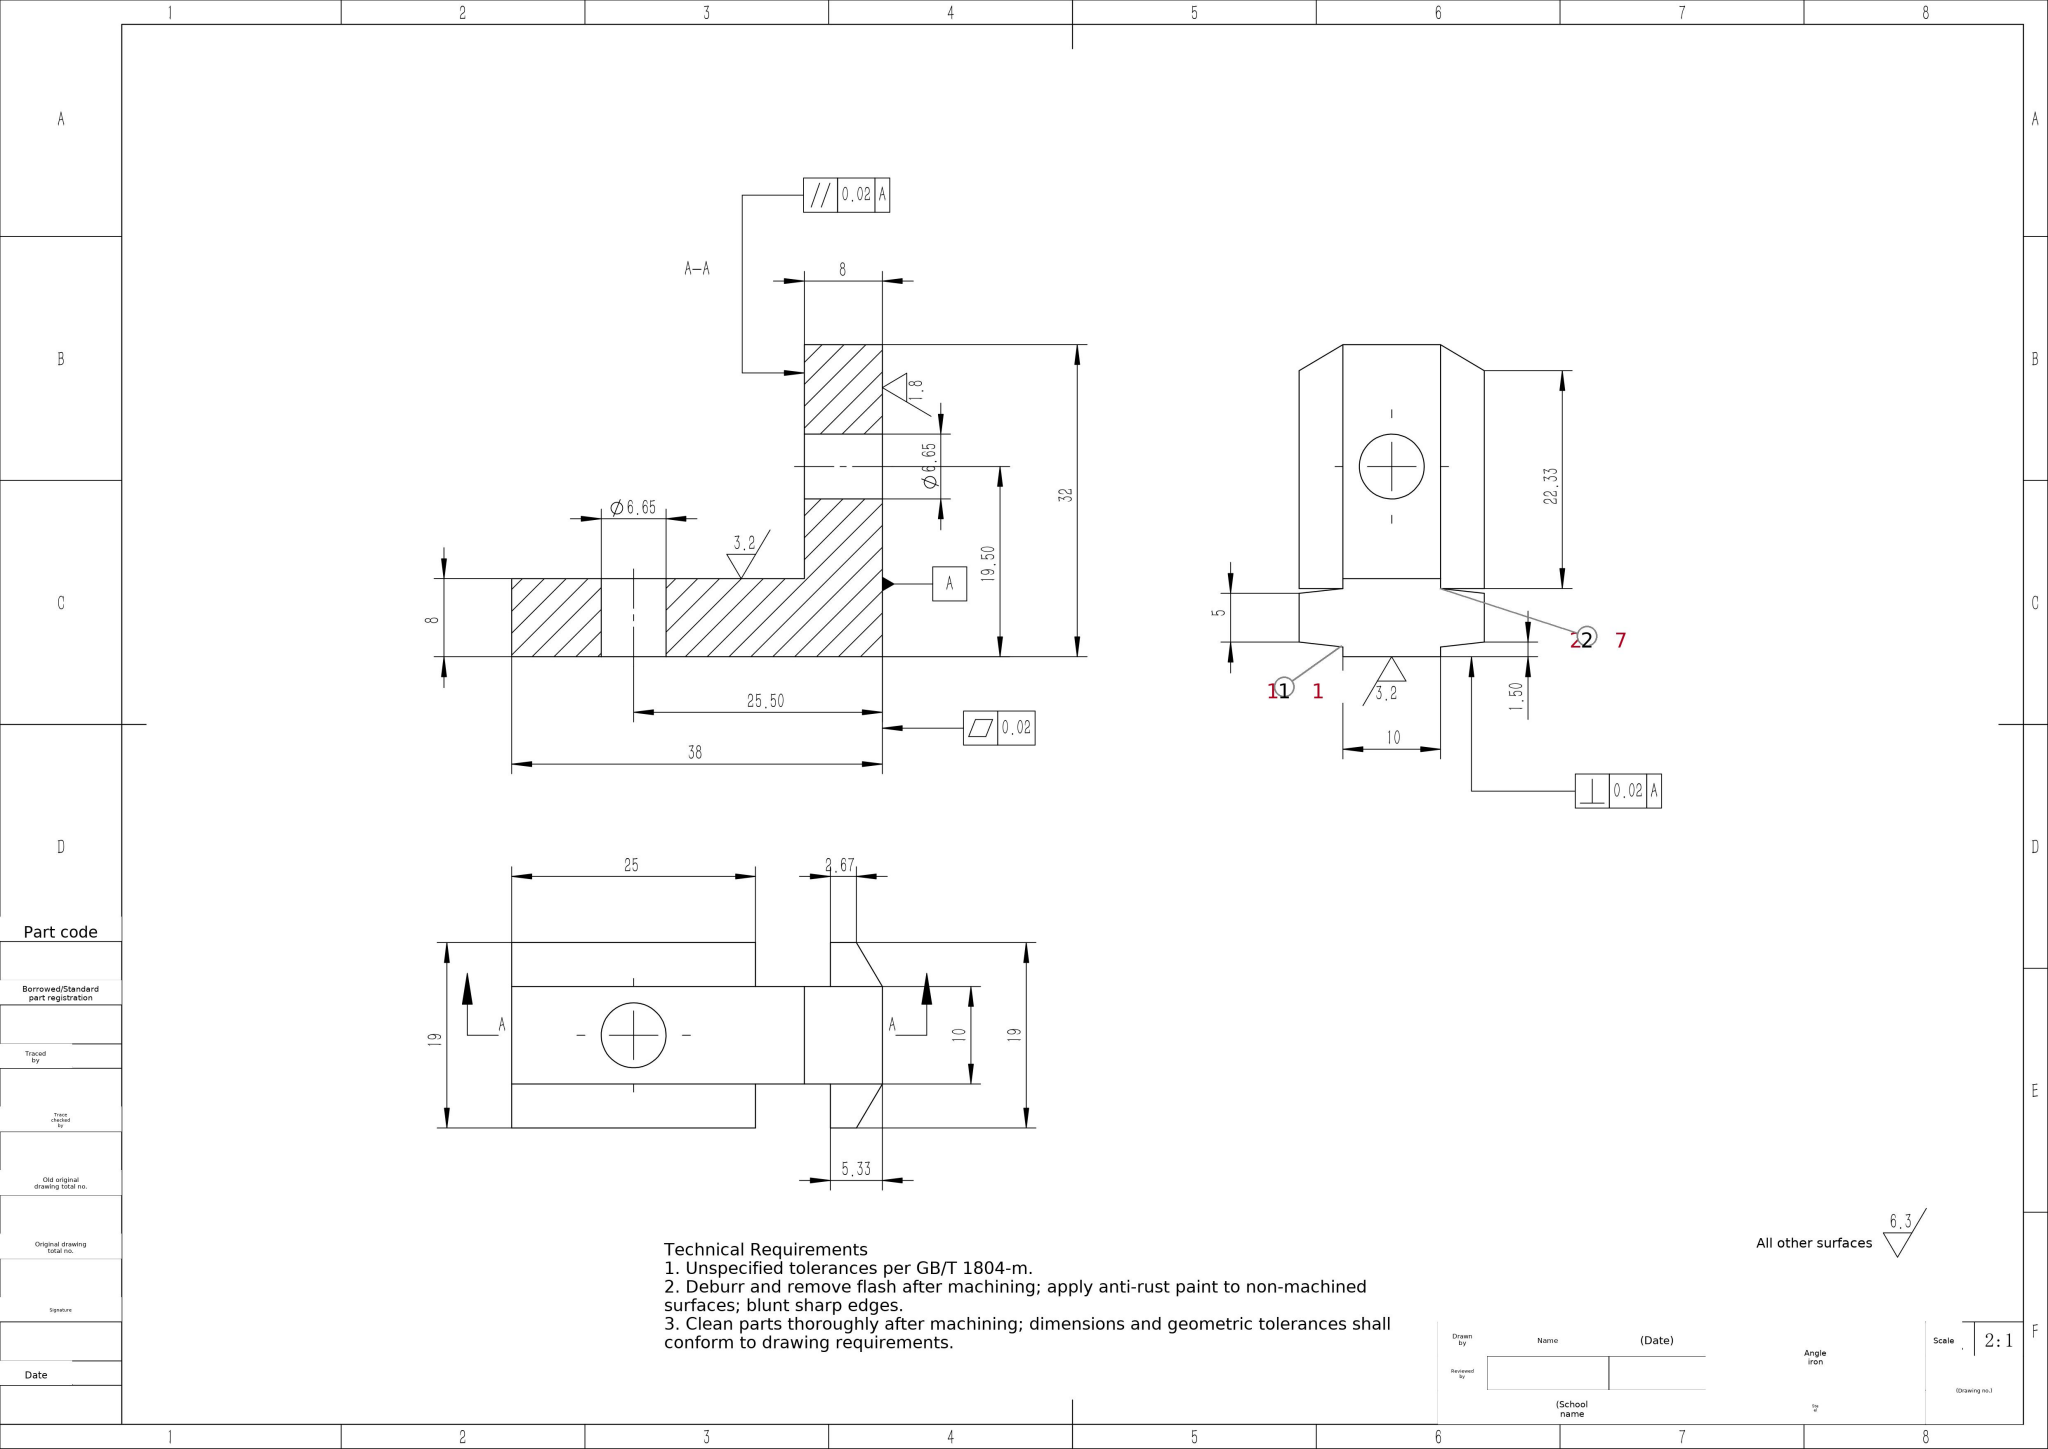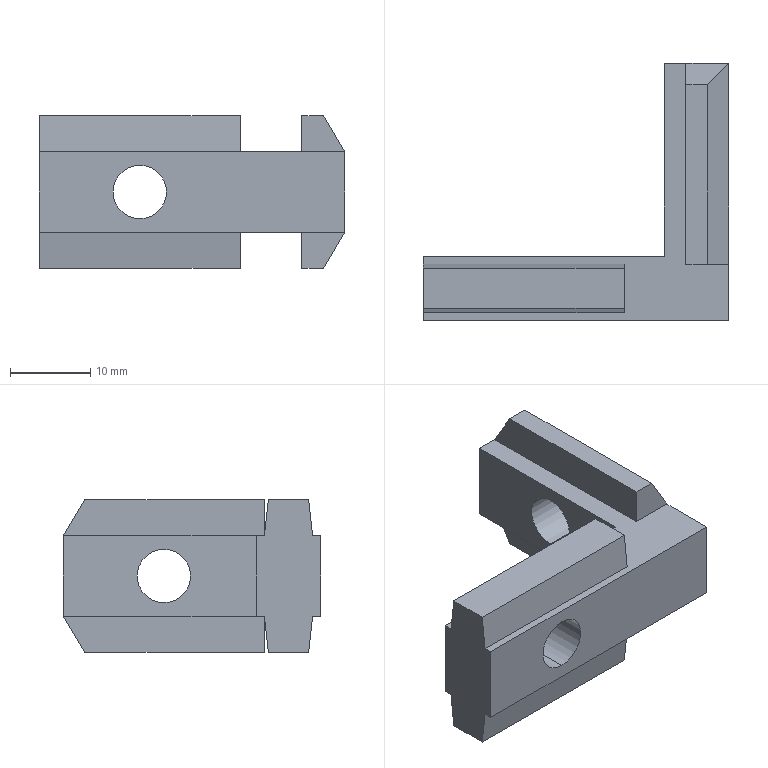Part | SolidWorks | mm | 1 solid | 30 faces | box 38 x 32 x 19 mm | volume 6500 mm3 | plane 26 | cylinder 4 | commonest cylinder face diameters 6.647 x4
STEP:
#1=CARTESIAN_POINT('',(0.,19.5,-3.324));
#2=VERTEX_POINT('',#1);
#3=CARTESIAN_POINT('',(0.,19.5,3.323));
#4=VERTEX_POINT('',#3);
#5=CARTESIAN_POINT('',(0.,19.5,-0.));
#6=DIRECTION('',(-1.,0.,0.));
#7=DIRECTION('',(0.,0.,1.));
#8=AXIS2_PLACEMENT_3D('',#5,#6,#7);
#9=CIRCLE('',#8,3.323);
#10=EDGE_CURVE('',#2,#4,#9,.T.);
#11=ORIENTED_EDGE('',*,*,#10,.F.);
#12=CARTESIAN_POINT('',(-8.,19.5,-3.323));
#13=VERTEX_POINT('',#12);
#14=CARTESIAN_POINT('',(-8.,19.5,-3.323));
#15=DIRECTION('',(-1.,0.,0.));
#16=VECTOR('',#15,1000.);
#17=LINE('',#14,#16);
#18=EDGE_CURVE('',#2,#13,#17,.T.);
#19=ORIENTED_EDGE('',*,*,#18,.T.);
#20=CARTESIAN_POINT('',(-8.,19.5,3.323));
#21=VERTEX_POINT('',#20);
#22=CARTESIAN_POINT('',(-8.,19.5,0.));
#23=DIRECTION('',(-1.,0.,0.));
#24=DIRECTION('',(0.,0.,1.));
#25=AXIS2_PLACEMENT_3D('',#22,#23,#24);
#26=CIRCLE('',#25,3.323);
#27=EDGE_CURVE('',#13,#21,#26,.T.);
#28=ORIENTED_EDGE('',*,*,#27,.T.);
#29=CARTESIAN_POINT('',(-8.,19.5,3.323));
#30=DIRECTION('',(-1.,0.,0.));
#31=VECTOR('',#30,1000.);
#32=LINE('',#29,#31);
#33=EDGE_CURVE('',#4,#21,#32,.T.);
#34=ORIENTED_EDGE('',*,*,#33,.F.);
#35=EDGE_LOOP('',(#11,#19,#28,#34));
#36=FACE_OUTER_BOUND('',#35,.T.);
#37=CARTESIAN_POINT('',(-8.,19.5,0.));
#38=DIRECTION('',(-1.,0.,0.));
#39=DIRECTION('',(0.,0.,1.));
#40=AXIS2_PLACEMENT_3D('',#37,#38,#39);
#41=CYLINDRICAL_SURFACE('',#40,3.323);
#42=ADVANCED_FACE('',(#36),#41,.F.);
#43=CARTESIAN_POINT('',(-25.5,8.,3.323));
#44=VERTEX_POINT('',#43);
#45=CARTESIAN_POINT('',(-25.5,8.,-3.323));
#46=VERTEX_POINT('',#45);
#47=CARTESIAN_POINT('',(-25.5,8.,0.));
#48=DIRECTION('',(-0.,-1.,-0.));
#49=DIRECTION('',(0.,0.,-1.));
#50=AXIS2_PLACEMENT_3D('',#47,#48,#49);
#51=CIRCLE('',#50,3.323);
#52=EDGE_CURVE('',#44,#46,#51,.T.);
#53=ORIENTED_EDGE('',*,*,#52,.F.);
#54=CARTESIAN_POINT('',(-25.5,-0.,3.323));
#55=VERTEX_POINT('',#54);
#56=CARTESIAN_POINT('',(-25.5,0.,3.323));
#57=DIRECTION('',(0.,-1.,0.));
#58=VECTOR('',#57,1000.);
#59=LINE('',#56,#58);
#60=EDGE_CURVE('',#44,#55,#59,.T.);
#61=ORIENTED_EDGE('',*,*,#60,.T.);
#62=CARTESIAN_POINT('',(-25.5,-0.,-3.323));
#63=VERTEX_POINT('',#62);
#64=CARTESIAN_POINT('',(-25.5,-0.,0.));
#65=DIRECTION('',(0.,-1.,0.));
#66=DIRECTION('',(0.,0.,-1.));
#67=AXIS2_PLACEMENT_3D('',#64,#65,#66);
#68=CIRCLE('',#67,3.323);
#69=EDGE_CURVE('',#55,#63,#68,.T.);
#70=ORIENTED_EDGE('',*,*,#69,.T.);
#71=CARTESIAN_POINT('',(-25.5,0.,-3.323));
#72=DIRECTION('',(0.,-1.,0.));
#73=VECTOR('',#72,1000.);
#74=LINE('',#71,#73);
#75=EDGE_CURVE('',#46,#63,#74,.T.);
#76=ORIENTED_EDGE('',*,*,#75,.F.);
#77=EDGE_LOOP('',(#53,#61,#70,#76));
#78=FACE_OUTER_BOUND('',#77,.T.);
#79=CARTESIAN_POINT('',(-25.5,0.,0.));
#80=DIRECTION('',(0.,-1.,0.));
#81=DIRECTION('',(0.,0.,-1.));
#82=AXIS2_PLACEMENT_3D('',#79,#80,#81);
#83=CYLINDRICAL_SURFACE('',#82,3.323);
#84=ADVANCED_FACE('',(#78),#83,.F.);
#85=CARTESIAN_POINT('',(0.,7.,-5.));
#86=VERTEX_POINT('',#85);
#87=CARTESIAN_POINT('',(-5.333,7.,-5.));
#88=VERTEX_POINT('',#87);
#89=CARTESIAN_POINT('',(-5.333,7.,-5.));
#90=DIRECTION('',(-1.,0.,0.));
#91=VECTOR('',#90,1000.);
#92=LINE('',#89,#91);
#93=EDGE_CURVE('',#86,#88,#92,.T.);
#94=ORIENTED_EDGE('',*,*,#93,.F.);
#95=CARTESIAN_POINT('',(0.,0.,-5.));
#96=VERTEX_POINT('',#95);
#97=CARTESIAN_POINT('',(0.,32.,-5.));
#98=DIRECTION('',(0.,-1.,-0.));
#99=VECTOR('',#98,1000.);
#100=LINE('',#97,#99);
#101=EDGE_CURVE('',#86,#96,#100,.T.);
#102=ORIENTED_EDGE('',*,*,#101,.T.);
#103=CARTESIAN_POINT('',(-38.,0.,-5.));
#104=VERTEX_POINT('',#103);
#105=CARTESIAN_POINT('',(0.,0.,-5.));
#106=DIRECTION('',(1.,0.,0.));
#107=VECTOR('',#106,1000.);
#108=LINE('',#105,#107);
#109=EDGE_CURVE('',#104,#96,#108,.T.);
#110=ORIENTED_EDGE('',*,*,#109,.F.);
#111=CARTESIAN_POINT('',(-38.,1.,-5.));
#112=VERTEX_POINT('',#111);
#113=CARTESIAN_POINT('',(-38.,0.,-5.));
#114=DIRECTION('',(0.,1.,0.));
#115=VECTOR('',#114,1000.);
#116=LINE('',#113,#115);
#117=EDGE_CURVE('',#104,#112,#116,.T.);
#118=ORIENTED_EDGE('',*,*,#117,.T.);
#119=CARTESIAN_POINT('',(-13.,1.,-5.));
#120=VERTEX_POINT('',#119);
#121=CARTESIAN_POINT('',(-38.,1.,-5.));
#122=DIRECTION('',(1.,0.,0.));
#123=VECTOR('',#122,1000.);
#124=LINE('',#121,#123);
#125=EDGE_CURVE('',#112,#120,#124,.T.);
#126=ORIENTED_EDGE('',*,*,#125,.T.);
#127=CARTESIAN_POINT('',(-13.,7.,-5.));
#128=VERTEX_POINT('',#127);
#129=CARTESIAN_POINT('',(-13.,7.,-5.));
#130=DIRECTION('',(0.,-1.,0.));
#131=VECTOR('',#130,1000.);
#132=LINE('',#129,#131);
#133=EDGE_CURVE('',#128,#120,#132,.T.);
#134=ORIENTED_EDGE('',*,*,#133,.F.);
#135=CARTESIAN_POINT('',(-38.,7.,-5.));
#136=VERTEX_POINT('',#135);
#137=CARTESIAN_POINT('',(-38.,7.,-5.));
#138=DIRECTION('',(1.,0.,0.));
#139=VECTOR('',#138,1000.);
#140=LINE('',#137,#139);
#141=EDGE_CURVE('',#136,#128,#140,.T.);
#142=ORIENTED_EDGE('',*,*,#141,.F.);
#143=CARTESIAN_POINT('',(-38.,8.,-5.));
#144=VERTEX_POINT('',#143);
#145=CARTESIAN_POINT('',(-38.,32.,-5.));
#146=DIRECTION('',(0.,-1.,-0.));
#147=VECTOR('',#146,1000.);
#148=LINE('',#145,#147);
#149=EDGE_CURVE('',#144,#136,#148,.T.);
#150=ORIENTED_EDGE('',*,*,#149,.F.);
#151=CARTESIAN_POINT('',(-8.,8.,-5.));
#152=VERTEX_POINT('',#151);
#153=CARTESIAN_POINT('',(-8.,8.,-5.));
#154=DIRECTION('',(-1.,0.,0.));
#155=VECTOR('',#154,1000.);
#156=LINE('',#153,#155);
#157=EDGE_CURVE('',#152,#144,#156,.T.);
#158=ORIENTED_EDGE('',*,*,#157,.F.);
#159=CARTESIAN_POINT('',(-8.,32.,-5.));
#160=VERTEX_POINT('',#159);
#161=CARTESIAN_POINT('',(-8.,32.,-5.));
#162=DIRECTION('',(0.,-1.,-0.));
#163=VECTOR('',#162,1000.);
#164=LINE('',#161,#163);
#165=EDGE_CURVE('',#160,#152,#164,.T.);
#166=ORIENTED_EDGE('',*,*,#165,.F.);
#167=CARTESIAN_POINT('',(-5.333,32.,-5.));
#168=VERTEX_POINT('',#167);
#169=CARTESIAN_POINT('',(-38.,32.,-5.));
#170=DIRECTION('',(-1.,0.,0.));
#171=VECTOR('',#170,1000.);
#172=LINE('',#169,#171);
#173=EDGE_CURVE('',#168,#160,#172,.T.);
#174=ORIENTED_EDGE('',*,*,#173,.F.);
#175=CARTESIAN_POINT('',(-5.333,32.,-5.));
#176=DIRECTION('',(0.,1.,0.));
#177=VECTOR('',#176,1000.);
#178=LINE('',#175,#177);
#179=EDGE_CURVE('',#88,#168,#178,.T.);
#180=ORIENTED_EDGE('',*,*,#179,.F.);
#181=EDGE_LOOP('',(#94,#102,#110,#118,#126,#134,#142,#150,#158,#166,#174,#180));
#182=FACE_OUTER_BOUND('',#181,.T.);
#183=CARTESIAN_POINT('',(-38.,32.,-5.));
#184=DIRECTION('',(0.,-0.,1.));
#185=DIRECTION('',(1.,0.,-0.));
#186=AXIS2_PLACEMENT_3D('',#183,#184,#185);
#187=PLANE('',#186);
#188=ADVANCED_FACE('',(#182),#187,.F.);
#189=CARTESIAN_POINT('',(-5.333,32.,5.));
#190=VERTEX_POINT('',#189);
#191=CARTESIAN_POINT('',(-5.333,7.,5.));
#192=VERTEX_POINT('',#191);
#193=CARTESIAN_POINT('',(-5.333,7.,5.));
#194=DIRECTION('',(0.,-1.,0.));
#195=VECTOR('',#194,1000.);
#196=LINE('',#193,#195);
#197=EDGE_CURVE('',#190,#192,#196,.T.);
#198=ORIENTED_EDGE('',*,*,#197,.F.);
#199=CARTESIAN_POINT('',(-8.,32.,5.));
#200=VERTEX_POINT('',#199);
#201=CARTESIAN_POINT('',(0.,32.,5.));
#202=DIRECTION('',(1.,0.,0.));
#203=VECTOR('',#202,1000.);
#204=LINE('',#201,#203);
#205=EDGE_CURVE('',#200,#190,#204,.T.);
#206=ORIENTED_EDGE('',*,*,#205,.F.);
#207=CARTESIAN_POINT('',(-8.,8.,5.));
#208=VERTEX_POINT('',#207);
#209=CARTESIAN_POINT('',(-8.,32.,5.));
#210=DIRECTION('',(-0.,-1.,-0.));
#211=VECTOR('',#210,1000.);
#212=LINE('',#209,#211);
#213=EDGE_CURVE('',#200,#208,#212,.T.);
#214=ORIENTED_EDGE('',*,*,#213,.T.);
#215=CARTESIAN_POINT('',(-38.,8.,5.));
#216=VERTEX_POINT('',#215);
#217=CARTESIAN_POINT('',(0.,8.,5.));
#218=DIRECTION('',(-1.,0.,0.));
#219=VECTOR('',#218,1000.);
#220=LINE('',#217,#219);
#221=EDGE_CURVE('',#208,#216,#220,.T.);
#222=ORIENTED_EDGE('',*,*,#221,.T.);
#223=CARTESIAN_POINT('',(-38.,7.,5.));
#224=VERTEX_POINT('',#223);
#225=CARTESIAN_POINT('',(-38.,32.,5.));
#226=DIRECTION('',(0.,-1.,-0.));
#227=VECTOR('',#226,1000.);
#228=LINE('',#225,#227);
#229=EDGE_CURVE('',#216,#224,#228,.T.);
#230=ORIENTED_EDGE('',*,*,#229,.T.);
#231=CARTESIAN_POINT('',(-13.,7.,5.));
#232=VERTEX_POINT('',#231);
#233=CARTESIAN_POINT('',(-38.,7.,5.));
#234=DIRECTION('',(1.,0.,0.));
#235=VECTOR('',#234,1000.);
#236=LINE('',#233,#235);
#237=EDGE_CURVE('',#224,#232,#236,.T.);
#238=ORIENTED_EDGE('',*,*,#237,.T.);
#239=CARTESIAN_POINT('',(-13.,1.,5.));
#240=VERTEX_POINT('',#239);
#241=CARTESIAN_POINT('',(-13.,1.,5.));
#242=DIRECTION('',(-0.,1.,-0.));
#243=VECTOR('',#242,1000.);
#244=LINE('',#241,#243);
#245=EDGE_CURVE('',#240,#232,#244,.T.);
#246=ORIENTED_EDGE('',*,*,#245,.F.);
#247=CARTESIAN_POINT('',(-38.,1.,5.));
#248=VERTEX_POINT('',#247);
#249=CARTESIAN_POINT('',(-38.,1.,5.));
#250=DIRECTION('',(1.,0.,0.));
#251=VECTOR('',#250,1000.);
#252=LINE('',#249,#251);
#253=EDGE_CURVE('',#248,#240,#252,.T.);
#254=ORIENTED_EDGE('',*,*,#253,.F.);
#255=CARTESIAN_POINT('',(-38.,0.,5.));
#256=VERTEX_POINT('',#255);
#257=CARTESIAN_POINT('',(-38.,0.,5.));
#258=DIRECTION('',(0.,1.,0.));
#259=VECTOR('',#258,1000.);
#260=LINE('',#257,#259);
#261=EDGE_CURVE('',#256,#248,#260,.T.);
#262=ORIENTED_EDGE('',*,*,#261,.F.);
#263=CARTESIAN_POINT('',(0.,0.,5.));
#264=VERTEX_POINT('',#263);
#265=CARTESIAN_POINT('',(-38.,0.,5.));
#266=DIRECTION('',(-1.,0.,0.));
#267=VECTOR('',#266,1000.);
#268=LINE('',#265,#267);
#269=EDGE_CURVE('',#264,#256,#268,.T.);
#270=ORIENTED_EDGE('',*,*,#269,.F.);
#271=CARTESIAN_POINT('',(0.,7.,5.));
#272=VERTEX_POINT('',#271);
#273=CARTESIAN_POINT('',(0.,32.,5.));
#274=DIRECTION('',(0.,-1.,-0.));
#275=VECTOR('',#274,1000.);
#276=LINE('',#273,#275);
#277=EDGE_CURVE('',#272,#264,#276,.T.);
#278=ORIENTED_EDGE('',*,*,#277,.F.);
#279=CARTESIAN_POINT('',(0.,7.,5.));
#280=DIRECTION('',(1.,0.,0.));
#281=VECTOR('',#280,1000.);
#282=LINE('',#279,#281);
#283=EDGE_CURVE('',#192,#272,#282,.T.);
#284=ORIENTED_EDGE('',*,*,#283,.F.);
#285=EDGE_LOOP('',(#198,#206,#214,#222,#230,#238,#246,#254,#262,#270,#278,#284));
#286=FACE_OUTER_BOUND('',#285,.T.);
#287=CARTESIAN_POINT('',(0.,32.,5.));
#288=DIRECTION('',(0.,0.,-1.));
#289=DIRECTION('',(0.,1.,0.));
#290=AXIS2_PLACEMENT_3D('',#287,#288,#289);
#291=PLANE('',#290);
#292=ADVANCED_FACE('',(#286),#291,.F.);
#293=CARTESIAN_POINT('',(-38.,6.5,-9.5));
#294=VERTEX_POINT('',#293);
#295=CARTESIAN_POINT('',(-13.,6.5,-9.5));
#296=VERTEX_POINT('',#295);
#297=CARTESIAN_POINT('',(-38.,6.5,-9.5));
#298=DIRECTION('',(1.,0.,0.));
#299=VECTOR('',#298,1000.);
#300=LINE('',#297,#299);
#301=EDGE_CURVE('',#294,#296,#300,.T.);
#302=ORIENTED_EDGE('',*,*,#301,.T.);
#303=CARTESIAN_POINT('',(-13.,1.5,-9.5));
#304=VERTEX_POINT('',#303);
#305=CARTESIAN_POINT('',(-13.,1.5,-9.5));
#306=DIRECTION('',(-0.,1.,0.));
#307=VECTOR('',#306,1000.);
#308=LINE('',#305,#307);
#309=EDGE_CURVE('',#304,#296,#308,.T.);
#310=ORIENTED_EDGE('',*,*,#309,.F.);
#311=CARTESIAN_POINT('',(-38.,1.5,-9.5));
#312=VERTEX_POINT('',#311);
#313=CARTESIAN_POINT('',(-38.,1.5,-9.5));
#314=DIRECTION('',(1.,0.,0.));
#315=VECTOR('',#314,1000.);
#316=LINE('',#313,#315);
#317=EDGE_CURVE('',#312,#304,#316,.T.);
#318=ORIENTED_EDGE('',*,*,#317,.F.);
#319=CARTESIAN_POINT('',(-38.,1.5,-9.5));
#320=DIRECTION('',(0.,1.,0.));
#321=VECTOR('',#320,1000.);
#322=LINE('',#319,#321);
#323=EDGE_CURVE('',#312,#294,#322,.T.);
#324=ORIENTED_EDGE('',*,*,#323,.T.);
#325=EDGE_LOOP('',(#302,#310,#318,#324));
#326=FACE_OUTER_BOUND('',#325,.T.);
#327=CARTESIAN_POINT('',(-38.,1.5,-9.5));
#328=DIRECTION('',(0.,0.,-1.));
#329=DIRECTION('',(0.,1.,0.));
#330=AXIS2_PLACEMENT_3D('',#327,#328,#329);
#331=PLANE('',#330);
#332=ADVANCED_FACE('',(#326),#331,.T.);
#333=ORIENTED_EDGE('',*,*,#317,.T.);
#334=CARTESIAN_POINT('',(-13.,1.,-5.));
#335=DIRECTION('',(-0.,0.1104,-0.9939));
#336=VECTOR('',#335,1000.);
#337=LINE('',#334,#336);
#338=EDGE_CURVE('',#120,#304,#337,.T.);
#339=ORIENTED_EDGE('',*,*,#338,.F.);
#340=ORIENTED_EDGE('',*,*,#125,.F.);
#341=CARTESIAN_POINT('',(-38.,1.,-5.));
#342=DIRECTION('',(0.,0.1104,-0.9939));
#343=VECTOR('',#342,1000.);
#344=LINE('',#341,#343);
#345=EDGE_CURVE('',#112,#312,#344,.T.);
#346=ORIENTED_EDGE('',*,*,#345,.T.);
#347=EDGE_LOOP('',(#333,#339,#340,#346));
#348=FACE_OUTER_BOUND('',#347,.T.);
#349=CARTESIAN_POINT('',(-38.,1.,-5.));
#350=DIRECTION('',(0.,-0.9939,-0.1104));
#351=DIRECTION('',(0.,0.1104,-0.9939));
#352=AXIS2_PLACEMENT_3D('',#349,#350,#351);
#353=PLANE('',#352);
#354=ADVANCED_FACE('',(#348),#353,.T.);
#355=ORIENTED_EDGE('',*,*,#141,.T.);
#356=CARTESIAN_POINT('',(-13.,6.5,-9.5));
#357=DIRECTION('',(0.,0.1104,0.9939));
#358=VECTOR('',#357,1000.);
#359=LINE('',#356,#358);
#360=EDGE_CURVE('',#296,#128,#359,.T.);
#361=ORIENTED_EDGE('',*,*,#360,.F.);
#362=ORIENTED_EDGE('',*,*,#301,.F.);
#363=CARTESIAN_POINT('',(-38.,6.5,-9.5));
#364=DIRECTION('',(0.,0.1104,0.9939));
#365=VECTOR('',#364,1000.);
#366=LINE('',#363,#365);
#367=EDGE_CURVE('',#294,#136,#366,.T.);
#368=ORIENTED_EDGE('',*,*,#367,.T.);
#369=EDGE_LOOP('',(#355,#361,#362,#368));
#370=FACE_OUTER_BOUND('',#369,.T.);
#371=CARTESIAN_POINT('',(-38.,6.5,-9.5));
#372=DIRECTION('',(0.,0.9939,-0.1104));
#373=DIRECTION('',(0.,0.1104,0.9939));
#374=AXIS2_PLACEMENT_3D('',#371,#372,#373);
#375=PLANE('',#374);
#376=ADVANCED_FACE('',(#370),#375,.T.);
#377=ORIENTED_EDGE('',*,*,#253,.T.);
#378=CARTESIAN_POINT('',(-13.,1.5,9.5));
#379=VERTEX_POINT('',#378);
#380=CARTESIAN_POINT('',(-13.,1.5,9.5));
#381=DIRECTION('',(-0.,-0.1104,-0.9939));
#382=VECTOR('',#381,1000.);
#383=LINE('',#380,#382);
#384=EDGE_CURVE('',#379,#240,#383,.T.);
#385=ORIENTED_EDGE('',*,*,#384,.F.);
#386=CARTESIAN_POINT('',(-38.,1.5,9.5));
#387=VERTEX_POINT('',#386);
#388=CARTESIAN_POINT('',(-38.,1.5,9.5));
#389=DIRECTION('',(1.,0.,0.));
#390=VECTOR('',#389,1000.);
#391=LINE('',#388,#390);
#392=EDGE_CURVE('',#387,#379,#391,.T.);
#393=ORIENTED_EDGE('',*,*,#392,.F.);
#394=CARTESIAN_POINT('',(-38.,1.5,9.5));
#395=DIRECTION('',(0.,-0.1104,-0.9939));
#396=VECTOR('',#395,1000.);
#397=LINE('',#394,#396);
#398=EDGE_CURVE('',#387,#248,#397,.T.);
#399=ORIENTED_EDGE('',*,*,#398,.T.);
#400=EDGE_LOOP('',(#377,#385,#393,#399));
#401=FACE_OUTER_BOUND('',#400,.T.);
#402=CARTESIAN_POINT('',(-38.,1.5,9.5));
#403=DIRECTION('',(0.,-0.9939,0.1104));
#404=DIRECTION('',(0.,-0.1104,-0.9939));
#405=AXIS2_PLACEMENT_3D('',#402,#403,#404);
#406=PLANE('',#405);
#407=ADVANCED_FACE('',(#401),#406,.T.);
#408=ORIENTED_EDGE('',*,*,#392,.T.);
#409=CARTESIAN_POINT('',(-13.,6.5,9.5));
#410=VERTEX_POINT('',#409);
#411=CARTESIAN_POINT('',(-13.,6.5,9.5));
#412=DIRECTION('',(0.,-1.,-0.));
#413=VECTOR('',#412,1000.);
#414=LINE('',#411,#413);
#415=EDGE_CURVE('',#410,#379,#414,.T.);
#416=ORIENTED_EDGE('',*,*,#415,.F.);
#417=CARTESIAN_POINT('',(-38.,6.5,9.5));
#418=VERTEX_POINT('',#417);
#419=CARTESIAN_POINT('',(-38.,6.5,9.5));
#420=DIRECTION('',(1.,0.,0.));
#421=VECTOR('',#420,1000.);
#422=LINE('',#419,#421);
#423=EDGE_CURVE('',#418,#410,#422,.T.);
#424=ORIENTED_EDGE('',*,*,#423,.F.);
#425=CARTESIAN_POINT('',(-38.,6.5,9.5));
#426=DIRECTION('',(0.,-1.,-0.));
#427=VECTOR('',#426,1000.);
#428=LINE('',#425,#427);
#429=EDGE_CURVE('',#418,#387,#428,.T.);
#430=ORIENTED_EDGE('',*,*,#429,.T.);
#431=EDGE_LOOP('',(#408,#416,#424,#430));
#432=FACE_OUTER_BOUND('',#431,.T.);
#433=CARTESIAN_POINT('',(-38.,6.5,9.5));
#434=DIRECTION('',(0.,-0.,1.));
#435=DIRECTION('',(0.,-1.,-0.));
#436=AXIS2_PLACEMENT_3D('',#433,#434,#435);
#437=PLANE('',#436);
#438=ADVANCED_FACE('',(#432),#437,.T.);
#439=ORIENTED_EDGE('',*,*,#423,.T.);
#440=CARTESIAN_POINT('',(-13.,7.,5.));
#441=DIRECTION('',(0.,-0.1104,0.9939));
#442=VECTOR('',#441,1000.);
#443=LINE('',#440,#442);
#444=EDGE_CURVE('',#232,#410,#443,.T.);
#445=ORIENTED_EDGE('',*,*,#444,.F.);
#446=ORIENTED_EDGE('',*,*,#237,.F.);
#447=CARTESIAN_POINT('',(-38.,7.,5.));
#448=DIRECTION('',(0.,-0.1104,0.9939));
#449=VECTOR('',#448,1000.);
#450=LINE('',#447,#449);
#451=EDGE_CURVE('',#224,#418,#450,.T.);
#452=ORIENTED_EDGE('',*,*,#451,.T.);
#453=EDGE_LOOP('',(#439,#445,#446,#452));
#454=FACE_OUTER_BOUND('',#453,.T.);
#455=CARTESIAN_POINT('',(-38.,7.,5.));
#456=DIRECTION('',(0.,0.9939,0.1104));
#457=DIRECTION('',(0.,-0.1104,0.9939));
#458=AXIS2_PLACEMENT_3D('',#455,#456,#457);
#459=PLANE('',#458);
#460=ADVANCED_FACE('',(#454),#459,.T.);
#461=ORIENTED_EDGE('',*,*,#229,.F.);
#462=CARTESIAN_POINT('',(-38.,8.,9.5));
#463=DIRECTION('',(-0.,0.,-1.));
#464=VECTOR('',#463,1000.);
#465=LINE('',#462,#464);
#466=EDGE_CURVE('',#216,#144,#465,.T.);
#467=ORIENTED_EDGE('',*,*,#466,.T.);
#468=ORIENTED_EDGE('',*,*,#149,.T.);
#469=ORIENTED_EDGE('',*,*,#367,.F.);
#470=ORIENTED_EDGE('',*,*,#323,.F.);
#471=ORIENTED_EDGE('',*,*,#345,.F.);
#472=ORIENTED_EDGE('',*,*,#117,.F.);
#473=CARTESIAN_POINT('',(-38.,0.,-5.));
#474=DIRECTION('',(0.,0.,-1.));
#475=VECTOR('',#474,1000.);
#476=LINE('',#473,#475);
#477=EDGE_CURVE('',#256,#104,#476,.T.);
#478=ORIENTED_EDGE('',*,*,#477,.F.);
#479=ORIENTED_EDGE('',*,*,#261,.T.);
#480=ORIENTED_EDGE('',*,*,#398,.F.);
#481=ORIENTED_EDGE('',*,*,#429,.F.);
#482=ORIENTED_EDGE('',*,*,#451,.F.);
#483=EDGE_LOOP('',(#461,#467,#468,#469,#470,#471,#472,#478,#479,#480,#481,#482));
#484=FACE_OUTER_BOUND('',#483,.T.);
#485=CARTESIAN_POINT('',(-38.,0.,0.));
#486=DIRECTION('',(1.,0.,0.));
#487=DIRECTION('',(0.,0.,-1.));
#488=AXIS2_PLACEMENT_3D('',#485,#486,#487);
#489=PLANE('',#488);
#490=ADVANCED_FACE('',(#484),#489,.F.);
#491=CARTESIAN_POINT('',(0.,19.5,-0.));
#492=DIRECTION('',(-1.,0.,0.));
#493=DIRECTION('',(0.,0.,1.));
#494=AXIS2_PLACEMENT_3D('',#491,#492,#493);
#495=CIRCLE('',#494,3.323);
#496=EDGE_CURVE('',#4,#2,#495,.T.);
#497=ORIENTED_EDGE('',*,*,#496,.T.);
#498=ORIENTED_EDGE('',*,*,#10,.T.);
#499=EDGE_LOOP('',(#497,#498));
#500=FACE_BOUND('',#499,.T.);
#501=ORIENTED_EDGE('',*,*,#101,.F.);
#502=CARTESIAN_POINT('',(0.,32.,-5.));
#503=VERTEX_POINT('',#502);
#504=CARTESIAN_POINT('',(0.,32.,-5.));
#505=DIRECTION('',(0.,1.,0.));
#506=VECTOR('',#505,1000.);
#507=LINE('',#504,#506);
#508=EDGE_CURVE('',#86,#503,#507,.T.);
#509=ORIENTED_EDGE('',*,*,#508,.T.);
#510=CARTESIAN_POINT('',(0.,32.,5.));
#511=VERTEX_POINT('',#510);
#512=CARTESIAN_POINT('',(0.,32.,-5.));
#513=DIRECTION('',(0.,0.,-1.));
#514=VECTOR('',#513,1000.);
#515=LINE('',#512,#514);
#516=EDGE_CURVE('',#511,#503,#515,.T.);
#517=ORIENTED_EDGE('',*,*,#516,.F.);
#518=CARTESIAN_POINT('',(0.,7.,5.));
#519=DIRECTION('',(0.,-1.,0.));
#520=VECTOR('',#519,1000.);
#521=LINE('',#518,#520);
#522=EDGE_CURVE('',#511,#272,#521,.T.);
#523=ORIENTED_EDGE('',*,*,#522,.T.);
#524=ORIENTED_EDGE('',*,*,#277,.T.);
#525=CARTESIAN_POINT('',(0.,0.,5.));
#526=DIRECTION('',(0.,0.,1.));
#527=VECTOR('',#526,1000.);
#528=LINE('',#525,#527);
#529=EDGE_CURVE('',#96,#264,#528,.T.);
#530=ORIENTED_EDGE('',*,*,#529,.F.);
#531=EDGE_LOOP('',(#501,#509,#517,#523,#524,#530));
#532=FACE_OUTER_BOUND('',#531,.T.);
#533=CARTESIAN_POINT('',(0.,0.,0.));
#534=DIRECTION('',(1.,0.,0.));
#535=DIRECTION('',(0.,0.,-1.));
#536=AXIS2_PLACEMENT_3D('',#533,#534,#535);
#537=PLANE('',#536);
#538=ADVANCED_FACE('',(#500,#532),#537,.T.);
#539=ORIENTED_EDGE('',*,*,#516,.T.);
#540=CARTESIAN_POINT('',(-0.,32.,-5.));
#541=DIRECTION('',(-1.,-0.,0.));
#542=VECTOR('',#541,1000.);
#543=LINE('',#540,#542);
#544=EDGE_CURVE('',#503,#168,#543,.T.);
#545=ORIENTED_EDGE('',*,*,#544,.T.);
#546=ORIENTED_EDGE('',*,*,#173,.T.);
#547=CARTESIAN_POINT('',(-8.,32.,0.));
#548=DIRECTION('',(0.,-0.,1.));
#549=VECTOR('',#548,1000.);
#550=LINE('',#547,#549);
#551=EDGE_CURVE('',#160,#200,#550,.T.);
#552=ORIENTED_EDGE('',*,*,#551,.T.);
#553=ORIENTED_EDGE('',*,*,#205,.T.);
#554=CARTESIAN_POINT('',(0.,32.,5.));
#555=DIRECTION('',(1.,0.,0.));
#556=VECTOR('',#555,1000.);
#557=LINE('',#554,#556);
#558=EDGE_CURVE('',#190,#511,#557,.T.);
#559=ORIENTED_EDGE('',*,*,#558,.T.);
#560=EDGE_LOOP('',(#539,#545,#546,#552,#553,#559));
#561=FACE_OUTER_BOUND('',#560,.T.);
#562=CARTESIAN_POINT('',(0.,32.,0.));
#563=DIRECTION('',(0.,-1.,-0.));
#564=DIRECTION('',(0.,0.,-1.));
#565=AXIS2_PLACEMENT_3D('',#562,#563,#564);
#566=PLANE('',#565);
#567=ADVANCED_FACE('',(#561),#566,.F.);
#568=ORIENTED_EDGE('',*,*,#415,.T.);
#569=ORIENTED_EDGE('',*,*,#384,.T.);
#570=ORIENTED_EDGE('',*,*,#245,.T.);
#571=ORIENTED_EDGE('',*,*,#444,.T.);
#572=EDGE_LOOP('',(#568,#569,#570,#571));
#573=FACE_OUTER_BOUND('',#572,.T.);
#574=CARTESIAN_POINT('',(-13.,-0.,0.));
#575=DIRECTION('',(1.,0.,-0.));
#576=DIRECTION('',(-0.,0.,-1.));
#577=AXIS2_PLACEMENT_3D('',#574,#575,#576);
#578=PLANE('',#577);
#579=ADVANCED_FACE('',(#573),#578,.T.);
#580=ORIENTED_EDGE('',*,*,#133,.T.);
#581=ORIENTED_EDGE('',*,*,#338,.T.);
#582=ORIENTED_EDGE('',*,*,#309,.T.);
#583=ORIENTED_EDGE('',*,*,#360,.T.);
#584=EDGE_LOOP('',(#580,#581,#582,#583));
#585=FACE_OUTER_BOUND('',#584,.T.);
#586=CARTESIAN_POINT('',(-13.,-0.,0.));
#587=DIRECTION('',(1.,0.,-0.));
#588=DIRECTION('',(-0.,0.,-1.));
#589=AXIS2_PLACEMENT_3D('',#586,#587,#588);
#590=PLANE('',#589);
#591=ADVANCED_FACE('',(#585),#590,.T.);
#592=CARTESIAN_POINT('',(-25.5,-0.,0.));
#593=DIRECTION('',(0.,-1.,0.));
#594=DIRECTION('',(0.,0.,-1.));
#595=AXIS2_PLACEMENT_3D('',#592,#593,#594);
#596=CIRCLE('',#595,3.323);
#597=EDGE_CURVE('',#63,#55,#596,.T.);
#598=ORIENTED_EDGE('',*,*,#597,.F.);
#599=ORIENTED_EDGE('',*,*,#69,.F.);
#600=EDGE_LOOP('',(#598,#599));
#601=FACE_BOUND('',#600,.T.);
#602=ORIENTED_EDGE('',*,*,#269,.T.);
#603=ORIENTED_EDGE('',*,*,#477,.T.);
#604=ORIENTED_EDGE('',*,*,#109,.T.);
#605=ORIENTED_EDGE('',*,*,#529,.T.);
#606=EDGE_LOOP('',(#602,#603,#604,#605));
#607=FACE_OUTER_BOUND('',#606,.T.);
#608=CARTESIAN_POINT('',(0.,0.,0.));
#609=DIRECTION('',(0.,1.,0.));
#610=DIRECTION('',(0.,0.,1.));
#611=AXIS2_PLACEMENT_3D('',#608,#609,#610);
#612=PLANE('',#611);
#613=ADVANCED_FACE('',(#601,#607),#612,.F.);
#614=CARTESIAN_POINT('',(-25.5,8.,0.));
#615=DIRECTION('',(-0.,-1.,-0.));
#616=DIRECTION('',(0.,0.,-1.));
#617=AXIS2_PLACEMENT_3D('',#614,#615,#616);
#618=CIRCLE('',#617,3.323);
#619=EDGE_CURVE('',#46,#44,#618,.T.);
#620=ORIENTED_EDGE('',*,*,#619,.T.);
#621=ORIENTED_EDGE('',*,*,#52,.T.);
#622=EDGE_LOOP('',(#620,#621));
#623=FACE_BOUND('',#622,.T.);
#624=CARTESIAN_POINT('',(-8.,8.,9.5));
#625=DIRECTION('',(-0.,0.,-1.));
#626=VECTOR('',#625,1000.);
#627=LINE('',#624,#626);
#628=EDGE_CURVE('',#208,#152,#627,.T.);
#629=ORIENTED_EDGE('',*,*,#628,.T.);
#630=ORIENTED_EDGE('',*,*,#157,.T.);
#631=ORIENTED_EDGE('',*,*,#466,.F.);
#632=ORIENTED_EDGE('',*,*,#221,.F.);
#633=EDGE_LOOP('',(#629,#630,#631,#632));
#634=FACE_OUTER_BOUND('',#633,.T.);
#635=CARTESIAN_POINT('',(-8.,8.,9.5));
#636=DIRECTION('',(-0.,-1.,-0.));
#637=DIRECTION('',(0.,0.,-1.));
#638=AXIS2_PLACEMENT_3D('',#635,#636,#637);
#639=PLANE('',#638);
#640=ADVANCED_FACE('',(#623,#634),#639,.F.);
#641=CARTESIAN_POINT('',(-8.,19.5,0.));
#642=DIRECTION('',(-1.,0.,0.));
#643=DIRECTION('',(0.,0.,1.));
#644=AXIS2_PLACEMENT_3D('',#641,#642,#643);
#645=CIRCLE('',#644,3.323);
#646=EDGE_CURVE('',#21,#13,#645,.T.);
#647=ORIENTED_EDGE('',*,*,#646,.F.);
#648=ORIENTED_EDGE('',*,*,#27,.F.);
#649=EDGE_LOOP('',(#647,#648));
#650=FACE_BOUND('',#649,.T.);
#651=ORIENTED_EDGE('',*,*,#551,.F.);
#652=ORIENTED_EDGE('',*,*,#165,.T.);
#653=ORIENTED_EDGE('',*,*,#628,.F.);
#654=ORIENTED_EDGE('',*,*,#213,.F.);
#655=EDGE_LOOP('',(#651,#652,#653,#654));
#656=FACE_OUTER_BOUND('',#655,.T.);
#657=CARTESIAN_POINT('',(-8.,32.,9.5));
#658=DIRECTION('',(1.,0.,-0.));
#659=DIRECTION('',(-0.,0.,-1.));
#660=AXIS2_PLACEMENT_3D('',#657,#658,#659);
#661=PLANE('',#660);
#662=ADVANCED_FACE('',(#650,#656),#661,.F.);
#663=CARTESIAN_POINT('',(-5.333,29.333,9.5));
#664=VERTEX_POINT('',#663);
#665=CARTESIAN_POINT('',(-5.333,7.,9.5));
#666=VERTEX_POINT('',#665);
#667=CARTESIAN_POINT('',(-5.333,7.,9.5));
#668=DIRECTION('',(0.,-1.,0.));
#669=VECTOR('',#668,1000.);
#670=LINE('',#667,#669);
#671=EDGE_CURVE('',#664,#666,#670,.T.);
#672=ORIENTED_EDGE('',*,*,#671,.F.);
#673=CARTESIAN_POINT('',(-5.333,29.333,9.5));
#674=DIRECTION('',(0.,0.5098,-0.8603));
#675=VECTOR('',#674,1000.);
#676=LINE('',#673,#675);
#677=EDGE_CURVE('',#664,#190,#676,.T.);
#678=ORIENTED_EDGE('',*,*,#677,.T.);
#679=ORIENTED_EDGE('',*,*,#197,.T.);
#680=CARTESIAN_POINT('',(-5.333,7.,9.5));
#681=DIRECTION('',(0.,0.,-1.));
#682=VECTOR('',#681,1000.);
#683=LINE('',#680,#682);
#684=EDGE_CURVE('',#666,#192,#683,.T.);
#685=ORIENTED_EDGE('',*,*,#684,.F.);
#686=EDGE_LOOP('',(#672,#678,#679,#685));
#687=FACE_OUTER_BOUND('',#686,.T.);
#688=CARTESIAN_POINT('',(-5.333,7.,9.5));
#689=DIRECTION('',(1.,0.,0.));
#690=DIRECTION('',(0.,0.,-1.));
#691=AXIS2_PLACEMENT_3D('',#688,#689,#690);
#692=PLANE('',#691);
#693=ADVANCED_FACE('',(#687),#692,.F.);
#694=ORIENTED_EDGE('',*,*,#283,.T.);
#695=CARTESIAN_POINT('',(-2.667,7.,9.5));
#696=VERTEX_POINT('',#695);
#697=CARTESIAN_POINT('',(-2.667,7.,9.5));
#698=DIRECTION('',(-0.5098,0.,0.8603));
#699=VECTOR('',#698,1000.);
#700=LINE('',#697,#699);
#701=EDGE_CURVE('',#272,#696,#700,.T.);
#702=ORIENTED_EDGE('',*,*,#701,.T.);
#703=CARTESIAN_POINT('',(0.,7.,9.5));
#704=DIRECTION('',(1.,0.,0.));
#705=VECTOR('',#704,1000.);
#706=LINE('',#703,#705);
#707=EDGE_CURVE('',#666,#696,#706,.T.);
#708=ORIENTED_EDGE('',*,*,#707,.F.);
#709=ORIENTED_EDGE('',*,*,#684,.T.);
#710=EDGE_LOOP('',(#694,#702,#708,#709));
#711=FACE_OUTER_BOUND('',#710,.T.);
#712=CARTESIAN_POINT('',(0.,7.,9.5));
#713=DIRECTION('',(0.,1.,0.));
#714=DIRECTION('',(0.,0.,1.));
#715=AXIS2_PLACEMENT_3D('',#712,#713,#714);
#716=PLANE('',#715);
#717=ADVANCED_FACE('',(#711),#716,.F.);
#718=CARTESIAN_POINT('',(-2.667,29.333,9.5));
#719=VERTEX_POINT('',#718);
#720=CARTESIAN_POINT('',(-2.667,32.,9.5));
#721=DIRECTION('',(0.,1.,0.));
#722=VECTOR('',#721,1000.);
#723=LINE('',#720,#722);
#724=EDGE_CURVE('',#696,#719,#723,.T.);
#725=ORIENTED_EDGE('',*,*,#724,.T.);
#726=CARTESIAN_POINT('',(0.,29.333,9.5));
#727=DIRECTION('',(-1.,0.,0.));
#728=VECTOR('',#727,1000.);
#729=LINE('',#726,#728);
#730=EDGE_CURVE('',#719,#664,#729,.T.);
#731=ORIENTED_EDGE('',*,*,#730,.T.);
#732=ORIENTED_EDGE('',*,*,#671,.T.);
#733=ORIENTED_EDGE('',*,*,#707,.T.);
#734=EDGE_LOOP('',(#725,#731,#732,#733));
#735=FACE_OUTER_BOUND('',#734,.T.);
#736=CARTESIAN_POINT('',(0.,0.,9.5));
#737=DIRECTION('',(0.,0.,-1.));
#738=DIRECTION('',(-1.,0.,0.));
#739=AXIS2_PLACEMENT_3D('',#736,#737,#738);
#740=PLANE('',#739);
#741=ADVANCED_FACE('',(#735),#740,.F.);
#742=CARTESIAN_POINT('',(-2.667,7.,-9.5));
#743=VERTEX_POINT('',#742);
#744=CARTESIAN_POINT('',(-5.333,7.,-9.5));
#745=VERTEX_POINT('',#744);
#746=CARTESIAN_POINT('',(-5.333,7.,-9.5));
#747=DIRECTION('',(-1.,0.,0.));
#748=VECTOR('',#747,1000.);
#749=LINE('',#746,#748);
#750=EDGE_CURVE('',#743,#745,#749,.T.);
#751=ORIENTED_EDGE('',*,*,#750,.F.);
#752=CARTESIAN_POINT('',(-2.667,7.,-9.5));
#753=DIRECTION('',(0.5098,-0.,0.8603));
#754=VECTOR('',#753,1000.);
#755=LINE('',#752,#754);
#756=EDGE_CURVE('',#743,#86,#755,.T.);
#757=ORIENTED_EDGE('',*,*,#756,.T.);
#758=ORIENTED_EDGE('',*,*,#93,.T.);
#759=CARTESIAN_POINT('',(-5.333,7.,-9.5));
#760=DIRECTION('',(0.,-0.,1.));
#761=VECTOR('',#760,1000.);
#762=LINE('',#759,#761);
#763=EDGE_CURVE('',#745,#88,#762,.T.);
#764=ORIENTED_EDGE('',*,*,#763,.F.);
#765=EDGE_LOOP('',(#751,#757,#758,#764));
#766=FACE_OUTER_BOUND('',#765,.T.);
#767=CARTESIAN_POINT('',(-5.333,7.,-9.5));
#768=DIRECTION('',(0.,1.,0.));
#769=DIRECTION('',(0.,-0.,1.));
#770=AXIS2_PLACEMENT_3D('',#767,#768,#769);
#771=PLANE('',#770);
#772=ADVANCED_FACE('',(#766),#771,.F.);
#773=ORIENTED_EDGE('',*,*,#179,.T.);
#774=CARTESIAN_POINT('',(-5.333,29.333,-9.5));
#775=VERTEX_POINT('',#774);
#776=CARTESIAN_POINT('',(-5.333,29.333,-9.5));
#777=DIRECTION('',(-0.,-0.5098,-0.8603));
#778=VECTOR('',#777,1000.);
#779=LINE('',#776,#778);
#780=EDGE_CURVE('',#168,#775,#779,.T.);
#781=ORIENTED_EDGE('',*,*,#780,.T.);
#782=CARTESIAN_POINT('',(-5.333,32.,-9.5));
#783=DIRECTION('',(0.,1.,0.));
#784=VECTOR('',#783,1000.);
#785=LINE('',#782,#784);
#786=EDGE_CURVE('',#745,#775,#785,.T.);
#787=ORIENTED_EDGE('',*,*,#786,.F.);
#788=ORIENTED_EDGE('',*,*,#763,.T.);
#789=EDGE_LOOP('',(#773,#781,#787,#788));
#790=FACE_OUTER_BOUND('',#789,.T.);
#791=CARTESIAN_POINT('',(-5.333,32.,-9.5));
#792=DIRECTION('',(1.,0.,-0.));
#793=DIRECTION('',(-0.,0.,-1.));
#794=AXIS2_PLACEMENT_3D('',#791,#792,#793);
#795=PLANE('',#794);
#796=ADVANCED_FACE('',(#790),#795,.F.);
#797=ORIENTED_EDGE('',*,*,#786,.T.);
#798=CARTESIAN_POINT('',(-2.667,29.333,-9.5));
#799=VERTEX_POINT('',#798);
#800=CARTESIAN_POINT('',(-0.,29.333,-9.5));
#801=DIRECTION('',(1.,0.,-0.));
#802=VECTOR('',#801,1000.);
#803=LINE('',#800,#802);
#804=EDGE_CURVE('',#775,#799,#803,.T.);
#805=ORIENTED_EDGE('',*,*,#804,.T.);
#806=CARTESIAN_POINT('',(-2.667,7.,-9.5));
#807=DIRECTION('',(0.,-1.,-0.));
#808=VECTOR('',#807,1000.);
#809=LINE('',#806,#808);
#810=EDGE_CURVE('',#799,#743,#809,.T.);
#811=ORIENTED_EDGE('',*,*,#810,.T.);
#812=ORIENTED_EDGE('',*,*,#750,.T.);
#813=EDGE_LOOP('',(#797,#805,#811,#812));
#814=FACE_OUTER_BOUND('',#813,.T.);
#815=CARTESIAN_POINT('',(-0.,0.,-9.5));
#816=DIRECTION('',(0.,-0.,1.));
#817=DIRECTION('',(1.,0.,-0.));
#818=AXIS2_PLACEMENT_3D('',#815,#816,#817);
#819=PLANE('',#818);
#820=ADVANCED_FACE('',(#814),#819,.F.);
#821=ORIENTED_EDGE('',*,*,#60,.F.);
#822=ORIENTED_EDGE('',*,*,#619,.F.);
#823=ORIENTED_EDGE('',*,*,#75,.T.);
#824=ORIENTED_EDGE('',*,*,#597,.T.);
#825=EDGE_LOOP('',(#821,#822,#823,#824));
#826=FACE_OUTER_BOUND('',#825,.T.);
#827=CARTESIAN_POINT('',(-25.5,0.,0.));
#828=DIRECTION('',(0.,-1.,0.));
#829=DIRECTION('',(0.,0.,-1.));
#830=AXIS2_PLACEMENT_3D('',#827,#828,#829);
#831=CYLINDRICAL_SURFACE('',#830,3.323);
#832=ADVANCED_FACE('',(#826),#831,.F.);
#833=ORIENTED_EDGE('',*,*,#18,.F.);
#834=ORIENTED_EDGE('',*,*,#496,.F.);
#835=ORIENTED_EDGE('',*,*,#33,.T.);
#836=ORIENTED_EDGE('',*,*,#646,.T.);
#837=EDGE_LOOP('',(#833,#834,#835,#836));
#838=FACE_OUTER_BOUND('',#837,.T.);
#839=CARTESIAN_POINT('',(-8.,19.5,0.));
#840=DIRECTION('',(-1.,0.,0.));
#841=DIRECTION('',(0.,0.,1.));
#842=AXIS2_PLACEMENT_3D('',#839,#840,#841);
#843=CYLINDRICAL_SURFACE('',#842,3.323);
#844=ADVANCED_FACE('',(#838),#843,.F.);
#845=ORIENTED_EDGE('',*,*,#701,.F.);
#846=ORIENTED_EDGE('',*,*,#522,.F.);
#847=CARTESIAN_POINT('',(-8.718,23.282,19.711));
#848=DIRECTION('',(0.4542,0.4542,-0.7664));
#849=VECTOR('',#848,1000.);
#850=LINE('',#847,#849);
#851=EDGE_CURVE('',#719,#511,#850,.T.);
#852=ORIENTED_EDGE('',*,*,#851,.F.);
#853=ORIENTED_EDGE('',*,*,#724,.F.);
#854=EDGE_LOOP('',(#845,#846,#852,#853));
#855=FACE_OUTER_BOUND('',#854,.T.);
#856=CARTESIAN_POINT('',(-2.667,0.,9.5));
#857=DIRECTION('',(0.8603,0.,0.5098));
#858=DIRECTION('',(0.,-1.,0.));
#859=AXIS2_PLACEMENT_3D('',#856,#857,#858);
#860=PLANE('',#859);
#861=ADVANCED_FACE('',(#855),#860,.T.);
#862=ORIENTED_EDGE('',*,*,#851,.T.);
#863=ORIENTED_EDGE('',*,*,#558,.F.);
#864=ORIENTED_EDGE('',*,*,#677,.F.);
#865=ORIENTED_EDGE('',*,*,#730,.F.);
#866=EDGE_LOOP('',(#862,#863,#864,#865));
#867=FACE_OUTER_BOUND('',#866,.T.);
#868=CARTESIAN_POINT('',(0.,29.333,9.5));
#869=DIRECTION('',(0.,-0.8603,-0.5098));
#870=DIRECTION('',(-1.,0.,0.));
#871=AXIS2_PLACEMENT_3D('',#868,#869,#870);
#872=PLANE('',#871);
#873=ADVANCED_FACE('',(#867),#872,.F.);
#874=ORIENTED_EDGE('',*,*,#756,.F.);
#875=ORIENTED_EDGE('',*,*,#810,.F.);
#876=CARTESIAN_POINT('',(-8.718,23.282,-19.711));
#877=DIRECTION('',(-0.4542,-0.4542,-0.7664));
#878=VECTOR('',#877,1000.);
#879=LINE('',#876,#878);
#880=EDGE_CURVE('',#503,#799,#879,.T.);
#881=ORIENTED_EDGE('',*,*,#880,.F.);
#882=ORIENTED_EDGE('',*,*,#508,.F.);
#883=EDGE_LOOP('',(#874,#875,#881,#882));
#884=FACE_OUTER_BOUND('',#883,.T.);
#885=CARTESIAN_POINT('',(-2.667,0.,-9.5));
#886=DIRECTION('',(0.8603,0.,-0.5098));
#887=DIRECTION('',(0.,1.,0.));
#888=AXIS2_PLACEMENT_3D('',#885,#886,#887);
#889=PLANE('',#888);
#890=ADVANCED_FACE('',(#884),#889,.T.);
#891=ORIENTED_EDGE('',*,*,#780,.F.);
#892=ORIENTED_EDGE('',*,*,#544,.F.);
#893=ORIENTED_EDGE('',*,*,#880,.T.);
#894=ORIENTED_EDGE('',*,*,#804,.F.);
#895=EDGE_LOOP('',(#891,#892,#893,#894));
#896=FACE_OUTER_BOUND('',#895,.T.);
#897=CARTESIAN_POINT('',(-0.,29.333,-9.5));
#898=DIRECTION('',(0.,-0.8603,0.5098));
#899=DIRECTION('',(1.,0.,-0.));
#900=AXIS2_PLACEMENT_3D('',#897,#898,#899);
#901=PLANE('',#900);
#902=ADVANCED_FACE('',(#896),#901,.F.);
#903=CLOSED_SHELL('',(#42,#84,#188,#292,#332,#354,#376,#407,#438,#460,#490,#538,#567,#579,#591,#613,#640,#662,#693,#717,#741,#772,#796,#820,#832,#844,#861,#873,#890,#902));
#904=MANIFOLD_SOLID_BREP('',#903);
#905=CARTESIAN_POINT('',(0.,0.,0.));
#906=DIRECTION('',(0.,0.,1.));
#907=DIRECTION('',(1.,0.,0.));
#908=AXIS2_PLACEMENT_3D('',#905,#906,#907);
#909=(LENGTH_UNIT()NAMED_UNIT(*)SI_UNIT(.MILLI.,.METRE.));
#910=UNCERTAINTY_MEASURE_WITH_UNIT(LENGTH_MEASURE(0.00001),#909,'','');
#911=(NAMED_UNIT(*)PLANE_ANGLE_UNIT()SI_UNIT($,.RADIAN.));
#912=(NAMED_UNIT(*)SI_UNIT($,.STERADIAN.)SOLID_ANGLE_UNIT());
#913=(GEOMETRIC_REPRESENTATION_CONTEXT(3)GLOBAL_UNCERTAINTY_ASSIGNED_CONTEXT((#910))GLOBAL_UNIT_ASSIGNED_CONTEXT((#909,#911,#912))REPRESENTATION_CONTEXT('',''));
#914=ADVANCED_BREP_SHAPE_REPRESENTATION('',(#904,#908),#913);